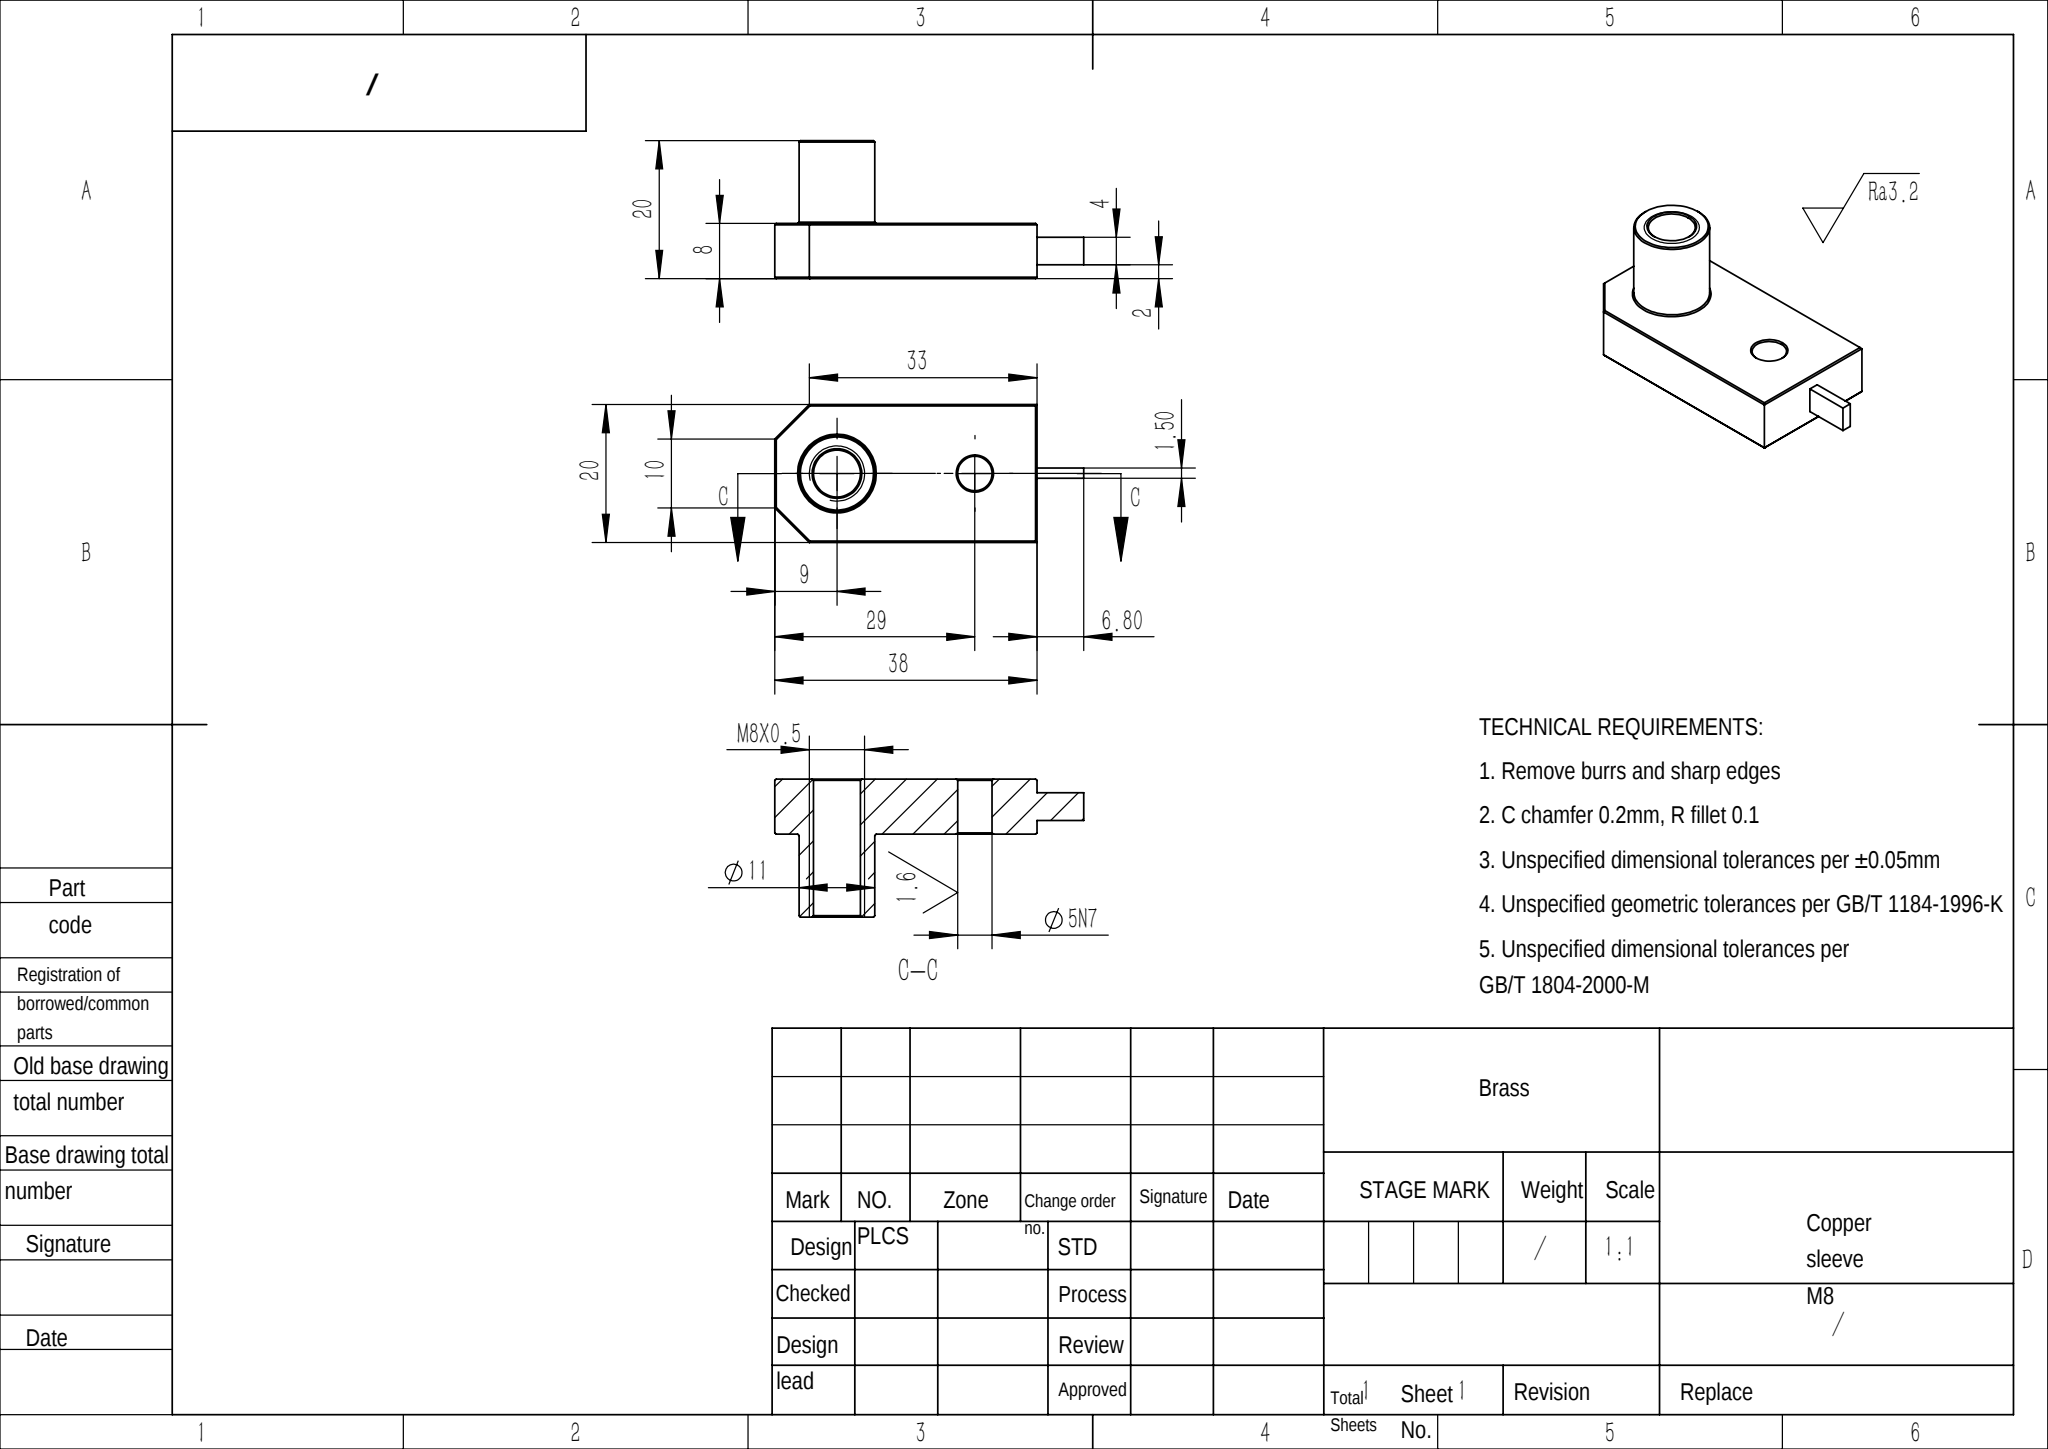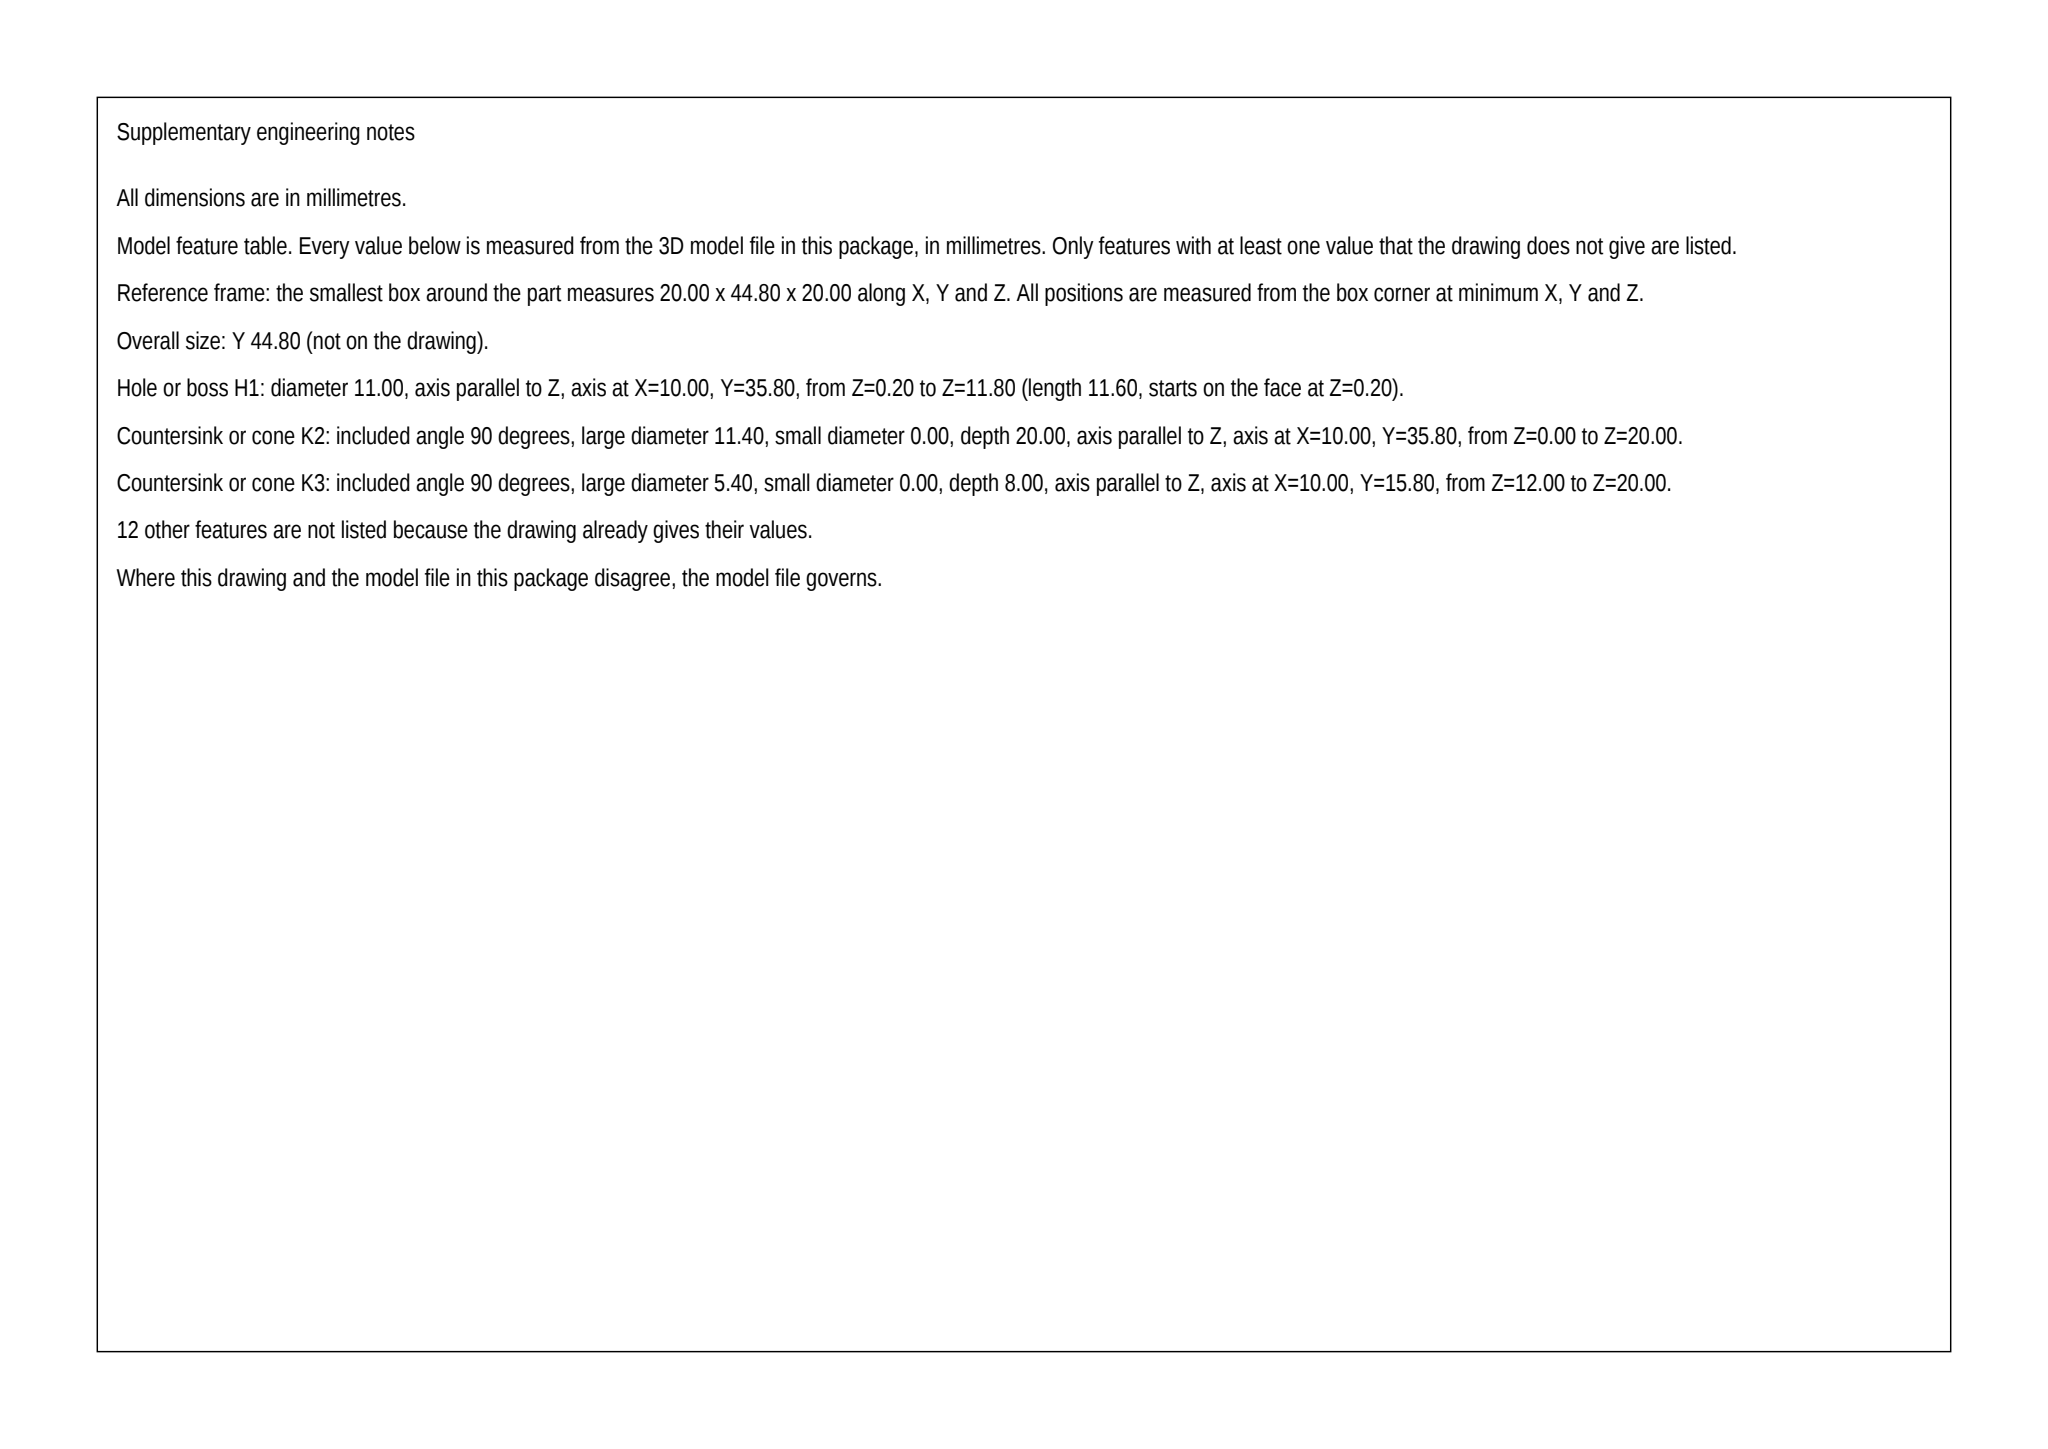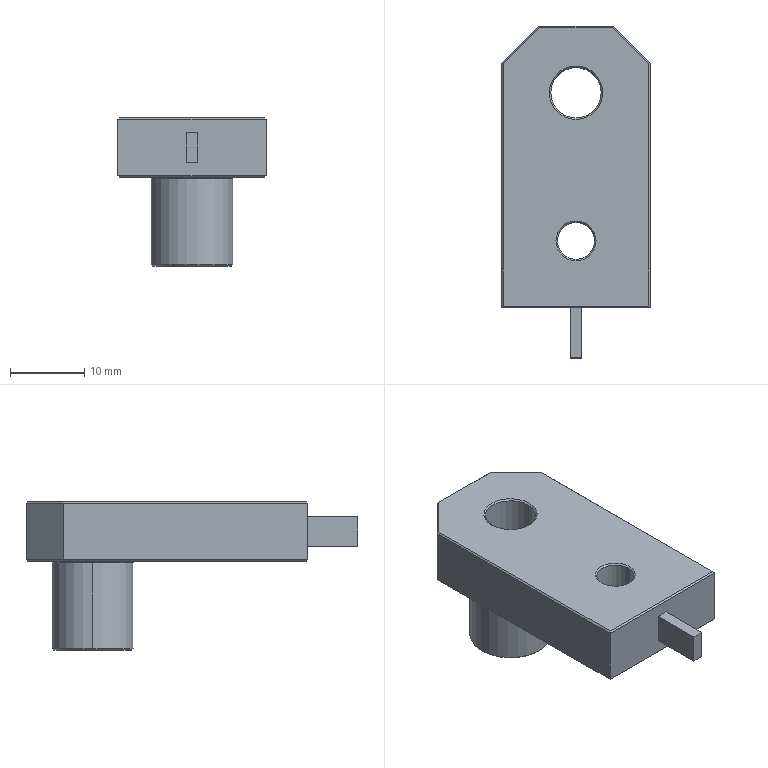Part | SolidWorks | mm | material Brass | 1 solid | 44 faces | box 20 x 44.8 x 20 mm | volume 6172 mm3 | plane 26 | cone 12 | cylinder 6 | commonest cylinder face diameters 6.8 x2 5 x2 11 x2